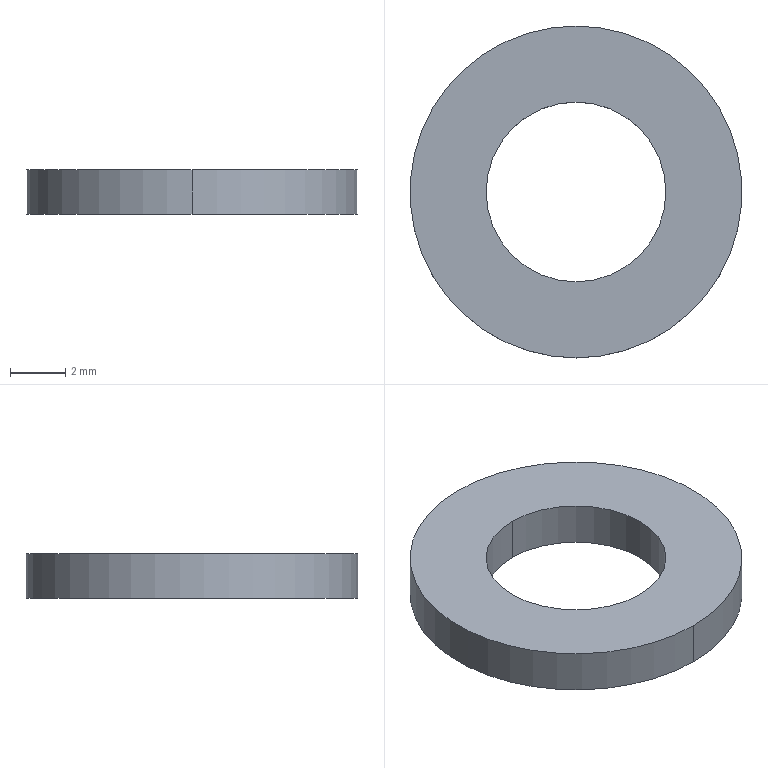Component | SolidWorks | FlatWasherCGrade6_1.6[GB_T95-2002]-10 | 1 solid | 6 faces | box 12 x 12 x 1.6 mm | volume 128 mm3 | cylinder 4 | plane 2 | commonest cylinder face diameters 12 x2 6.5 x2
build123d program:
from build123d import *

# Parameters (mm, degrees)
SKETCH1_W = 2.75
SKETCH1_H = 1.6


with BuildPart() as part:
    # Sketch1 → Base-Revolve (revolve)
    with BuildSketch(Plane.XY, mode=Mode.PRIVATE) as base_revolve_sk:
        with Locations((-4.625, 9.445)):
            Rectangle(SKETCH1_W, SKETCH1_H)
    revolve(base_revolve_sk.sketch.rotate(Axis((0, 0, 0), (0, 1, 0)), 270), axis=Axis((0, 0, 0), (0, 1, 0)))


solid = part.part

# Placed as in the assembly
solid = solid.moved(Location((75.494, 22.5, 9.355), (90, 0, 0)))
STEP:
#1=CARTESIAN_POINT('',(2.972,1.122,0.7717));
#2=VERTEX_POINT('',#1);
#3=CARTESIAN_POINT('',(2.972,0.6496,0.7717));
#4=VERTEX_POINT('',#3);
#5=CARTESIAN_POINT('',(2.972,0.8858,0.7717));
#6=DIRECTION('',(0.,0.,-1.));
#7=DIRECTION('',(0.,1.,0.));
#8=AXIS2_PLACEMENT_3D('',#5,#6,#7);
#9=CIRCLE('',#8,0.2362);
#10=EDGE_CURVE('',#2,#4,#9,.T.);
#11=ORIENTED_EDGE('',*,*,#10,.T.);
#12=CARTESIAN_POINT('',(2.972,0.6496,0.7087));
#13=VERTEX_POINT('',#12);
#14=CARTESIAN_POINT('',(2.972,0.6496,0.3683));
#15=DIRECTION('',(0.,0.,-1.));
#16=VECTOR('',#15,39.37);
#17=LINE('',#14,#16);
#18=EDGE_CURVE('',#4,#13,#17,.T.);
#19=ORIENTED_EDGE('',*,*,#18,.T.);
#20=CARTESIAN_POINT('',(2.972,1.122,0.7087));
#21=VERTEX_POINT('',#20);
#22=CARTESIAN_POINT('',(2.972,0.8858,0.7087));
#23=DIRECTION('',(0.,0.,-1.));
#24=DIRECTION('',(0.,1.,0.));
#25=AXIS2_PLACEMENT_3D('',#22,#23,#24);
#26=CIRCLE('',#25,0.2362);
#27=EDGE_CURVE('',#21,#13,#26,.T.);
#28=ORIENTED_EDGE('',*,*,#27,.F.);
#29=CARTESIAN_POINT('',(2.972,1.122,0.3683));
#30=DIRECTION('',(0.,0.,-1.));
#31=VECTOR('',#30,39.37);
#32=LINE('',#29,#31);
#33=EDGE_CURVE('',#2,#21,#32,.T.);
#34=ORIENTED_EDGE('',*,*,#33,.F.);
#35=EDGE_LOOP('',(#11,#19,#28,#34));
#36=FACE_OUTER_BOUND('',#35,.T.);
#37=CARTESIAN_POINT('',(2.972,0.8858,0.3683));
#38=DIRECTION('',(0.,0.,-1.));
#39=DIRECTION('',(0.,1.,0.));
#40=AXIS2_PLACEMENT_3D('',#37,#38,#39);
#41=CYLINDRICAL_SURFACE('',#40,0.2362);
#42=ADVANCED_FACE('',(#36),#41,.T.);
#43=CARTESIAN_POINT('',(2.972,0.7579,0.7717));
#44=VERTEX_POINT('',#43);
#45=CARTESIAN_POINT('',(2.972,1.014,0.7717));
#46=VERTEX_POINT('',#45);
#47=CARTESIAN_POINT('',(2.972,0.8858,0.7717));
#48=DIRECTION('',(0.,0.,-1.));
#49=DIRECTION('',(0.,1.,0.));
#50=AXIS2_PLACEMENT_3D('',#47,#48,#49);
#51=CIRCLE('',#50,0.128);
#52=EDGE_CURVE('',#44,#46,#51,.T.);
#53=ORIENTED_EDGE('',*,*,#52,.F.);
#54=CARTESIAN_POINT('',(2.972,0.7579,0.7087));
#55=VERTEX_POINT('',#54);
#56=CARTESIAN_POINT('',(2.972,0.7579,0.3683));
#57=DIRECTION('',(0.,0.,-1.));
#58=VECTOR('',#57,39.37);
#59=LINE('',#56,#58);
#60=EDGE_CURVE('',#44,#55,#59,.T.);
#61=ORIENTED_EDGE('',*,*,#60,.T.);
#62=CARTESIAN_POINT('',(2.972,1.014,0.7087));
#63=VERTEX_POINT('',#62);
#64=CARTESIAN_POINT('',(2.972,0.8858,0.7087));
#65=DIRECTION('',(0.,0.,-1.));
#66=DIRECTION('',(0.,1.,0.));
#67=AXIS2_PLACEMENT_3D('',#64,#65,#66);
#68=CIRCLE('',#67,0.128);
#69=EDGE_CURVE('',#55,#63,#68,.T.);
#70=ORIENTED_EDGE('',*,*,#69,.T.);
#71=CARTESIAN_POINT('',(2.972,1.014,0.3683));
#72=DIRECTION('',(0.,0.,-1.));
#73=VECTOR('',#72,39.37);
#74=LINE('',#71,#73);
#75=EDGE_CURVE('',#46,#63,#74,.T.);
#76=ORIENTED_EDGE('',*,*,#75,.F.);
#77=EDGE_LOOP('',(#53,#61,#70,#76));
#78=FACE_OUTER_BOUND('',#77,.T.);
#79=CARTESIAN_POINT('',(2.972,0.8858,0.3683));
#80=DIRECTION('',(0.,0.,-1.));
#81=DIRECTION('',(0.,1.,0.));
#82=AXIS2_PLACEMENT_3D('',#79,#80,#81);
#83=CYLINDRICAL_SURFACE('',#82,0.128);
#84=ADVANCED_FACE('',(#78),#83,.F.);
#85=ORIENTED_EDGE('',*,*,#60,.F.);
#86=CARTESIAN_POINT('',(2.972,0.8858,0.7717));
#87=DIRECTION('',(0.,0.,-1.));
#88=DIRECTION('',(0.,1.,0.));
#89=AXIS2_PLACEMENT_3D('',#86,#87,#88);
#90=CIRCLE('',#89,0.128);
#91=EDGE_CURVE('',#46,#44,#90,.T.);
#92=ORIENTED_EDGE('',*,*,#91,.F.);
#93=ORIENTED_EDGE('',*,*,#75,.T.);
#94=CARTESIAN_POINT('',(2.972,0.8858,0.7087));
#95=DIRECTION('',(0.,0.,-1.));
#96=DIRECTION('',(0.,1.,0.));
#97=AXIS2_PLACEMENT_3D('',#94,#95,#96);
#98=CIRCLE('',#97,0.128);
#99=EDGE_CURVE('',#63,#55,#98,.T.);
#100=ORIENTED_EDGE('',*,*,#99,.T.);
#101=EDGE_LOOP('',(#85,#92,#93,#100));
#102=FACE_OUTER_BOUND('',#101,.T.);
#103=CARTESIAN_POINT('',(2.972,0.8858,0.3683));
#104=DIRECTION('',(0.,0.,-1.));
#105=DIRECTION('',(0.,1.,0.));
#106=AXIS2_PLACEMENT_3D('',#103,#104,#105);
#107=CYLINDRICAL_SURFACE('',#106,0.128);
#108=ADVANCED_FACE('',(#102),#107,.F.);
#109=ORIENTED_EDGE('',*,*,#10,.F.);
#110=CARTESIAN_POINT('',(2.972,0.8858,0.7717));
#111=DIRECTION('',(0.,0.,-1.));
#112=DIRECTION('',(0.,1.,0.));
#113=AXIS2_PLACEMENT_3D('',#110,#111,#112);
#114=CIRCLE('',#113,0.2362);
#115=EDGE_CURVE('',#4,#2,#114,.T.);
#116=ORIENTED_EDGE('',*,*,#115,.F.);
#117=EDGE_LOOP('',(#109,#116));
#118=FACE_OUTER_BOUND('',#117,.T.);
#119=ORIENTED_EDGE('',*,*,#91,.T.);
#120=ORIENTED_EDGE('',*,*,#52,.T.);
#121=EDGE_LOOP('',(#119,#120));
#122=FACE_BOUND('',#121,.T.);
#123=CARTESIAN_POINT('',(2.844,0.8858,0.7717));
#124=DIRECTION('',(0.,0.,-1.));
#125=DIRECTION('',(0.,1.,0.));
#126=AXIS2_PLACEMENT_3D('',#123,#124,#125);
#127=PLANE('',#126);
#128=ADVANCED_FACE('',(#118,#122),#127,.F.);
#129=ORIENTED_EDGE('',*,*,#18,.F.);
#130=ORIENTED_EDGE('',*,*,#115,.T.);
#131=ORIENTED_EDGE('',*,*,#33,.T.);
#132=CARTESIAN_POINT('',(2.972,0.8858,0.7087));
#133=DIRECTION('',(0.,0.,-1.));
#134=DIRECTION('',(0.,1.,0.));
#135=AXIS2_PLACEMENT_3D('',#132,#133,#134);
#136=CIRCLE('',#135,0.2362);
#137=EDGE_CURVE('',#13,#21,#136,.T.);
#138=ORIENTED_EDGE('',*,*,#137,.F.);
#139=EDGE_LOOP('',(#129,#130,#131,#138));
#140=FACE_OUTER_BOUND('',#139,.T.);
#141=CARTESIAN_POINT('',(2.972,0.8858,0.3683));
#142=DIRECTION('',(0.,0.,-1.));
#143=DIRECTION('',(0.,1.,0.));
#144=AXIS2_PLACEMENT_3D('',#141,#142,#143);
#145=CYLINDRICAL_SURFACE('',#144,0.2362);
#146=ADVANCED_FACE('',(#140),#145,.T.);
#147=ORIENTED_EDGE('',*,*,#99,.F.);
#148=ORIENTED_EDGE('',*,*,#69,.F.);
#149=EDGE_LOOP('',(#147,#148));
#150=FACE_BOUND('',#149,.T.);
#151=ORIENTED_EDGE('',*,*,#27,.T.);
#152=ORIENTED_EDGE('',*,*,#137,.T.);
#153=EDGE_LOOP('',(#151,#152));
#154=FACE_OUTER_BOUND('',#153,.T.);
#155=CARTESIAN_POINT('',(2.844,0.8858,0.7087));
#156=DIRECTION('',(0.,0.,1.));
#157=DIRECTION('',(0.,-1.,0.));
#158=AXIS2_PLACEMENT_3D('',#155,#156,#157);
#159=PLANE('',#158);
#160=ADVANCED_FACE('',(#150,#154),#159,.F.);
#161=CLOSED_SHELL('',(#42,#84,#108,#128,#146,#160));
#162=MANIFOLD_SOLID_BREP('',#161);
#163=CARTESIAN_POINT('',(0.,0.,0.));
#164=DIRECTION('',(0.,0.,1.));
#165=DIRECTION('',(1.,0.,0.));
#166=AXIS2_PLACEMENT_3D('',#163,#164,#165);
#167=(LENGTH_UNIT()NAMED_UNIT(*)SI_UNIT($,.METRE.));
#168=LENGTH_MEASURE_WITH_UNIT(LENGTH_MEASURE(0.0254),#167);
#169=DIMENSIONAL_EXPONENTS(1.,0.,0.,0.,0.,0.,0.);
#170=(CONVERSION_BASED_UNIT('',#168)LENGTH_UNIT()NAMED_UNIT(#169));
#171=UNCERTAINTY_MEASURE_WITH_UNIT(LENGTH_MEASURE(0.00001),#170,'','');
#172=(NAMED_UNIT(*)PLANE_ANGLE_UNIT()SI_UNIT($,.RADIAN.));
#173=(NAMED_UNIT(*)SI_UNIT($,.STERADIAN.)SOLID_ANGLE_UNIT());
#174=(GEOMETRIC_REPRESENTATION_CONTEXT(3)GLOBAL_UNCERTAINTY_ASSIGNED_CONTEXT((#171))GLOBAL_UNIT_ASSIGNED_CONTEXT((#170,#172,#173))REPRESENTATION_CONTEXT('',''));
#175=ADVANCED_BREP_SHAPE_REPRESENTATION('',(#162,#166),#174);
#176=COLOUR_RGB('',0.7922,0.8196,0.9333);
#177=FILL_AREA_STYLE_COLOUR('',#176);
#178=FILL_AREA_STYLE('',(#177));
#179=SURFACE_STYLE_FILL_AREA(#178);
#180=SURFACE_SIDE_STYLE('',(#179));
#181=SURFACE_STYLE_USAGE(.BOTH.,#180);
#182=PRESENTATION_STYLE_ASSIGNMENT((#181));
#183=STYLED_ITEM('',(#182),#162);
#184=(LENGTH_UNIT()NAMED_UNIT(*)SI_UNIT($,.METRE.));
#185=LENGTH_MEASURE_WITH_UNIT(LENGTH_MEASURE(0.0254),#184);
#186=DIMENSIONAL_EXPONENTS(1.,0.,0.,0.,0.,0.,0.);
#187=(CONVERSION_BASED_UNIT('',#185)LENGTH_UNIT()NAMED_UNIT(#186));
#188=UNCERTAINTY_MEASURE_WITH_UNIT(LENGTH_MEASURE(0.00001),#187,'','');
#189=(NAMED_UNIT(*)PLANE_ANGLE_UNIT()SI_UNIT($,.RADIAN.));
#190=(NAMED_UNIT(*)SI_UNIT($,.STERADIAN.)SOLID_ANGLE_UNIT());
#191=(GEOMETRIC_REPRESENTATION_CONTEXT(3)GLOBAL_UNCERTAINTY_ASSIGNED_CONTEXT((#188))GLOBAL_UNIT_ASSIGNED_CONTEXT((#187,#189,#190))REPRESENTATION_CONTEXT('',''));
#192=MECHANICAL_DESIGN_GEOMETRIC_PRESENTATION_REPRESENTATION('',(#183),#191);
#193=PRESENTATION_LAYER_ASSIGNMENT('','',(#183));